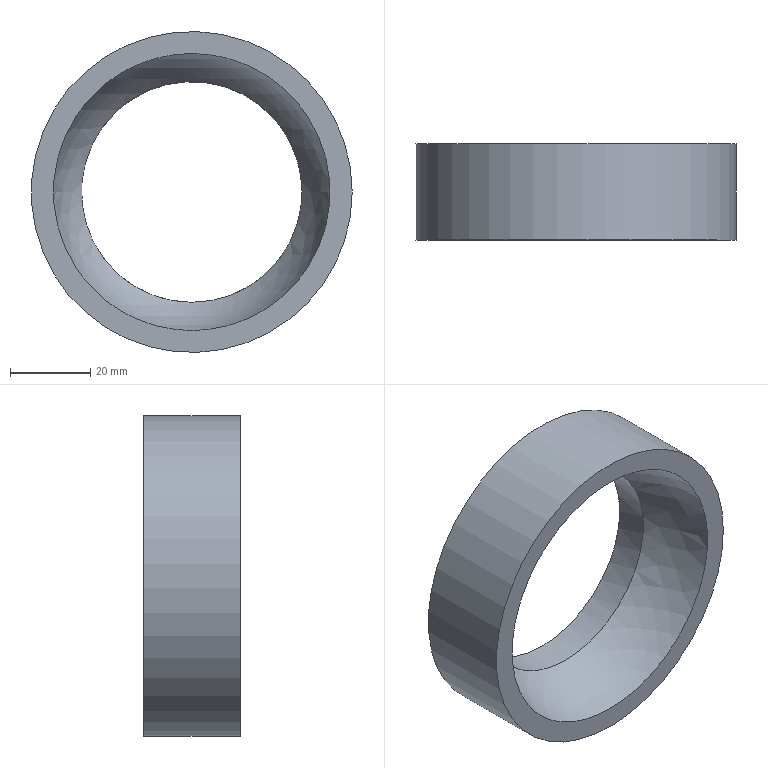Component | NX | MOVABLE_PAD | 1 solid | 5 faces | box 80 x 24 x 80 mm | volume 51017 mm3 | cylinder 2 | plane 2 | sphere 1 | commonest cylinder face diameters 80 x1 55 x1
STEP:
#1=CARTESIAN_POINT('',(0.,0.,0.));
#2=DIRECTION('',(0.,0.,1.));
#3=DIRECTION('',(1.,0.,0.));
#4=AXIS2_PLACEMENT_3D('',#1,#2,#3);
#5=CARTESIAN_POINT('',(223.939,30.,60.622));
#6=VERTEX_POINT('',#5);
#7=CARTESIAN_POINT('',(183.939,30.,60.622));
#8=DIRECTION('',(0.,-1.,0.));
#9=DIRECTION('',(1.,0.,0.));
#10=AXIS2_PLACEMENT_3D('',#7,#8,#9);
#11=CIRCLE('',#10,40.);
#12=CARTESIAN_POINT('',(183.939,30.,60.622));
#13=DIRECTION('',(0.,-1.,0.));
#14=DIRECTION('',(0.,0.,-1.));
#15=AXIS2_PLACEMENT_3D('',#12,#13,#14);
#16=CYLINDRICAL_SURFACE('',#15,40.);
#17=CARTESIAN_POINT('',(1.571,0.));
#18=DIRECTION('',(1.,0.));
#19=VECTOR('',#18,1.);
#20=LINE('',#17,#19);
#21=(GEOMETRIC_REPRESENTATION_CONTEXT(2)PARAMETRIC_REPRESENTATION_CONTEXT()REPRESENTATION_CONTEXT('',''));
#22=DEFINITIONAL_REPRESENTATION('',(#20),#21);
#23=PCURVE('',#16,#22);
#24=CARTESIAN_POINT('',(183.939,30.,60.622));
#25=DIRECTION('',(0.,-1.,0.));
#26=DIRECTION('',(0.,0.,-1.));
#27=AXIS2_PLACEMENT_3D('',#24,#25,#26);
#28=PLANE('',#27);
#29=CARTESIAN_POINT('',(0.,0.));
#30=DIRECTION('',(0.,1.));
#31=AXIS2_PLACEMENT_2D('',#29,#30);
#32=CIRCLE('',#31,40.);
#33=(GEOMETRIC_REPRESENTATION_CONTEXT(2)PARAMETRIC_REPRESENTATION_CONTEXT()REPRESENTATION_CONTEXT('',''));
#34=DEFINITIONAL_REPRESENTATION('',(#32),#33);
#35=PCURVE('',#28,#34);
#36=SURFACE_CURVE('',#11,(#23,#35),.PCURVE_S1.);
#37=EDGE_CURVE('',#6,#6,#36,.T.);
#38=ORIENTED_EDGE('',*,*,#37,.T.);
#39=CARTESIAN_POINT('',(223.939,6.,60.622));
#40=VERTEX_POINT('',#39);
#41=CARTESIAN_POINT('',(223.939,30.,60.622));
#42=CARTESIAN_POINT('',(223.939,6.,60.622));
#43=B_SPLINE_CURVE_WITH_KNOTS('',1,(#41,#42),.UNSPECIFIED.,.F.,.F.,(2,2),(0.,24.),.PIECEWISE_BEZIER_KNOTS.);
#44=CARTESIAN_POINT('',(7.854,0.));
#45=DIRECTION('',(0.,1.));
#46=VECTOR('',#45,1.);
#47=LINE('',#44,#46);
#48=(GEOMETRIC_REPRESENTATION_CONTEXT(2)PARAMETRIC_REPRESENTATION_CONTEXT()REPRESENTATION_CONTEXT('',''));
#49=DEFINITIONAL_REPRESENTATION('',(#47),#48);
#50=PCURVE('',#16,#49);
#51=CARTESIAN_POINT('',(1.571,0.));
#52=DIRECTION('',(0.,1.));
#53=VECTOR('',#52,1.);
#54=LINE('',#51,#53);
#55=(GEOMETRIC_REPRESENTATION_CONTEXT(2)PARAMETRIC_REPRESENTATION_CONTEXT()REPRESENTATION_CONTEXT('',''));
#56=DEFINITIONAL_REPRESENTATION('',(#54),#55);
#57=PCURVE('',#16,#56);
#58=SEAM_CURVE('',#43,(#50,#57),.PCURVE_S1.);
#59=EDGE_CURVE('',#6,#40,#58,.T.);
#60=ORIENTED_EDGE('',*,*,#59,.T.);
#61=CARTESIAN_POINT('',(183.939,6.,60.622));
#62=DIRECTION('',(0.,-1.,0.));
#63=DIRECTION('',(1.,0.,0.));
#64=AXIS2_PLACEMENT_3D('',#61,#62,#63);
#65=CIRCLE('',#64,40.);
#66=CARTESIAN_POINT('',(1.571,24.));
#67=DIRECTION('',(1.,0.));
#68=VECTOR('',#67,1.);
#69=LINE('',#66,#68);
#70=(GEOMETRIC_REPRESENTATION_CONTEXT(2)PARAMETRIC_REPRESENTATION_CONTEXT()REPRESENTATION_CONTEXT('',''));
#71=DEFINITIONAL_REPRESENTATION('',(#69),#70);
#72=PCURVE('',#16,#71);
#73=CARTESIAN_POINT('',(183.939,6.,60.622));
#74=DIRECTION('',(0.,-1.,0.));
#75=DIRECTION('',(0.,0.,-1.));
#76=AXIS2_PLACEMENT_3D('',#73,#74,#75);
#77=PLANE('',#76);
#78=CARTESIAN_POINT('',(0.,0.));
#79=DIRECTION('',(0.,1.));
#80=AXIS2_PLACEMENT_2D('',#78,#79);
#81=CIRCLE('',#80,40.);
#82=(GEOMETRIC_REPRESENTATION_CONTEXT(2)PARAMETRIC_REPRESENTATION_CONTEXT()REPRESENTATION_CONTEXT('',''));
#83=DEFINITIONAL_REPRESENTATION('',(#81),#82);
#84=PCURVE('',#77,#83);
#85=SURFACE_CURVE('',#65,(#72,#84),.PCURVE_S1.);
#86=EDGE_CURVE('',#40,#40,#85,.T.);
#87=ORIENTED_EDGE('',*,*,#86,.F.);
#88=ORIENTED_EDGE('',*,*,#59,.F.);
#89=EDGE_LOOP('',(#38,#60,#87,#88));
#90=FACE_BOUND('',#89,.T.);
#91=ADVANCED_FACE('',(#90),#16,.T.);
#92=CARTESIAN_POINT('',(183.939,21.651,33.122));
#93=VERTEX_POINT('',#92);
#94=CARTESIAN_POINT('',(183.939,21.651,60.622));
#95=DIRECTION('',(0.,-1.,0.));
#96=DIRECTION('',(0.,0.,-1.));
#97=AXIS2_PLACEMENT_3D('',#94,#95,#96);
#98=CIRCLE('',#97,27.5);
#99=CARTESIAN_POINT('',(183.939,30.,60.622));
#100=DIRECTION('',(0.,-1.,0.));
#101=DIRECTION('',(0.,0.,-1.));
#102=AXIS2_PLACEMENT_3D('',#99,#100,#101);
#103=CYLINDRICAL_SURFACE('',#102,27.5);
#104=CARTESIAN_POINT('',(0.,8.349));
#105=DIRECTION('',(1.,0.));
#106=VECTOR('',#105,1.);
#107=LINE('',#104,#106);
#108=(GEOMETRIC_REPRESENTATION_CONTEXT(2)PARAMETRIC_REPRESENTATION_CONTEXT()REPRESENTATION_CONTEXT('',''));
#109=DEFINITIONAL_REPRESENTATION('',(#107),#108);
#110=PCURVE('',#103,#109);
#111=CARTESIAN_POINT('',(183.939,-0.,60.622));
#112=DIRECTION('',(0.,0.,1.));
#113=DIRECTION('',(1.,0.,0.));
#114=AXIS2_PLACEMENT_3D('',#111,#112,#113);
#115=SPHERICAL_SURFACE('',#114,35.);
#116=CARTESIAN_POINT('',(1.571,-0.9038));
#117=CARTESIAN_POINT('',(1.443,-0.9044));
#118=CARTESIAN_POINT('',(1.213,-0.8677));
#119=CARTESIAN_POINT('',(0.9516,-0.7301));
#120=CARTESIAN_POINT('',(0.7946,-0.5446));
#121=CARTESIAN_POINT('',(0.7052,-0.3344));
#122=CARTESIAN_POINT('',(0.6653,-0.1126));
#123=CARTESIAN_POINT('',(0.6653,0.1126));
#124=CARTESIAN_POINT('',(0.7053,0.3344));
#125=CARTESIAN_POINT('',(0.7943,0.5446));
#126=CARTESIAN_POINT('',(0.9525,0.7301));
#127=CARTESIAN_POINT('',(1.21,0.868));
#128=CARTESIAN_POINT('',(1.571,0.9218));
#129=CARTESIAN_POINT('',(1.932,0.868));
#130=CARTESIAN_POINT('',(2.189,0.7301));
#131=CARTESIAN_POINT('',(2.347,0.5446));
#132=CARTESIAN_POINT('',(2.436,0.3344));
#133=CARTESIAN_POINT('',(2.476,0.1126));
#134=CARTESIAN_POINT('',(2.476,-0.1126));
#135=CARTESIAN_POINT('',(2.436,-0.3344));
#136=CARTESIAN_POINT('',(2.347,-0.5446));
#137=CARTESIAN_POINT('',(2.19,-0.7301));
#138=CARTESIAN_POINT('',(1.928,-0.8677));
#139=CARTESIAN_POINT('',(1.699,-0.9044));
#140=CARTESIAN_POINT('',(1.571,-0.9038));
#141=B_SPLINE_CURVE_WITH_KNOTS('',3,(#116,#117,#118,#119,#120,#121,#122,#123,#124,#125,#126,#127,#128,#129,#130,#131,#132,#133,#134,#135,#136,#137,#138,#139,#140),.UNSPECIFIED.,.T.,.F.,(4,1,1,1,1,1,1,1,1,1,1,1,1,1,1,1,1,1,1,1,1,1,4),(0.,0.2856,0.5712,0.8568,1.142,1.428,1.714,1.999,2.285,2.57,2.856,3.142,3.427,3.713,3.998,4.284,4.57,4.855,5.141,5.426,5.712,5.998,6.283),.QUASI_UNIFORM_KNOTS.);
#142=(GEOMETRIC_REPRESENTATION_CONTEXT(2)PARAMETRIC_REPRESENTATION_CONTEXT()REPRESENTATION_CONTEXT('',''));
#143=DEFINITIONAL_REPRESENTATION('',(#141),#142);
#144=PCURVE('',#115,#143);
#145=SURFACE_CURVE('',#98,(#110,#144),.PCURVE_S1.);
#146=EDGE_CURVE('',#93,#93,#145,.T.);
#147=ORIENTED_EDGE('',*,*,#146,.F.);
#148=CARTESIAN_POINT('',(183.939,30.,33.122));
#149=VERTEX_POINT('',#148);
#150=CARTESIAN_POINT('',(183.939,30.,33.122));
#151=CARTESIAN_POINT('',(183.939,21.651,33.122));
#152=B_SPLINE_CURVE_WITH_KNOTS('',1,(#150,#151),.UNSPECIFIED.,.F.,.F.,(2,2),(0.,8.349),.PIECEWISE_BEZIER_KNOTS.);
#153=CARTESIAN_POINT('',(0.,0.));
#154=DIRECTION('',(0.,1.));
#155=VECTOR('',#154,1.);
#156=LINE('',#153,#155);
#157=(GEOMETRIC_REPRESENTATION_CONTEXT(2)PARAMETRIC_REPRESENTATION_CONTEXT()REPRESENTATION_CONTEXT('',''));
#158=DEFINITIONAL_REPRESENTATION('',(#156),#157);
#159=PCURVE('',#103,#158);
#160=CARTESIAN_POINT('',(6.283,0.));
#161=DIRECTION('',(0.,1.));
#162=VECTOR('',#161,1.);
#163=LINE('',#160,#162);
#164=(GEOMETRIC_REPRESENTATION_CONTEXT(2)PARAMETRIC_REPRESENTATION_CONTEXT()REPRESENTATION_CONTEXT('',''));
#165=DEFINITIONAL_REPRESENTATION('',(#163),#164);
#166=PCURVE('',#103,#165);
#167=SEAM_CURVE('',#152,(#159,#166),.PCURVE_S1.);
#168=EDGE_CURVE('',#149,#93,#167,.T.);
#169=ORIENTED_EDGE('',*,*,#168,.F.);
#170=CARTESIAN_POINT('',(211.439,30.,60.622));
#171=VERTEX_POINT('',#170);
#172=CARTESIAN_POINT('',(183.939,30.,60.622));
#173=DIRECTION('',(0.,-1.,0.));
#174=DIRECTION('',(1.,0.,0.));
#175=AXIS2_PLACEMENT_3D('',#172,#173,#174);
#176=CIRCLE('',#175,27.5);
#177=CARTESIAN_POINT('',(-4.712,0.));
#178=DIRECTION('',(1.,0.));
#179=VECTOR('',#178,1.);
#180=LINE('',#177,#179);
#181=(GEOMETRIC_REPRESENTATION_CONTEXT(2)PARAMETRIC_REPRESENTATION_CONTEXT()REPRESENTATION_CONTEXT('',''));
#182=DEFINITIONAL_REPRESENTATION('',(#180),#181);
#183=PCURVE('',#103,#182);
#184=CARTESIAN_POINT('',(0.,0.));
#185=DIRECTION('',(0.,1.));
#186=AXIS2_PLACEMENT_2D('',#184,#185);
#187=CIRCLE('',#186,27.5);
#188=(GEOMETRIC_REPRESENTATION_CONTEXT(2)PARAMETRIC_REPRESENTATION_CONTEXT()REPRESENTATION_CONTEXT('',''));
#189=DEFINITIONAL_REPRESENTATION('',(#187),#188);
#190=PCURVE('',#28,#189);
#191=SURFACE_CURVE('',#176,(#183,#190),.PCURVE_S1.);
#192=EDGE_CURVE('',#149,#171,#191,.T.);
#193=ORIENTED_EDGE('',*,*,#192,.T.);
#194=CARTESIAN_POINT('',(183.939,30.,60.622));
#195=DIRECTION('',(0.,-1.,0.));
#196=DIRECTION('',(1.,0.,0.));
#197=AXIS2_PLACEMENT_3D('',#194,#195,#196);
#198=CIRCLE('',#197,27.5);
#199=CARTESIAN_POINT('',(1.571,0.));
#200=DIRECTION('',(1.,0.));
#201=VECTOR('',#200,1.);
#202=LINE('',#199,#201);
#203=(GEOMETRIC_REPRESENTATION_CONTEXT(2)PARAMETRIC_REPRESENTATION_CONTEXT()REPRESENTATION_CONTEXT('',''));
#204=DEFINITIONAL_REPRESENTATION('',(#202),#203);
#205=PCURVE('',#103,#204);
#206=CARTESIAN_POINT('',(0.,0.));
#207=DIRECTION('',(0.,1.));
#208=AXIS2_PLACEMENT_2D('',#206,#207);
#209=CIRCLE('',#208,27.5);
#210=(GEOMETRIC_REPRESENTATION_CONTEXT(2)PARAMETRIC_REPRESENTATION_CONTEXT()REPRESENTATION_CONTEXT('',''));
#211=DEFINITIONAL_REPRESENTATION('',(#209),#210);
#212=PCURVE('',#28,#211);
#213=SURFACE_CURVE('',#198,(#205,#212),.PCURVE_S1.);
#214=EDGE_CURVE('',#171,#149,#213,.T.);
#215=ORIENTED_EDGE('',*,*,#214,.T.);
#216=ORIENTED_EDGE('',*,*,#168,.T.);
#217=EDGE_LOOP('',(#147,#169,#193,#215,#216));
#218=FACE_BOUND('',#217,.F.);
#219=ADVANCED_FACE('',(#218),#103,.F.);
#220=ORIENTED_EDGE('',*,*,#37,.F.);
#221=EDGE_LOOP('',(#220));
#222=FACE_BOUND('',#221,.T.);
#223=ORIENTED_EDGE('',*,*,#214,.T.);
#224=ORIENTED_EDGE('',*,*,#192,.T.);
#225=EDGE_LOOP('',(#223,#224));
#226=FACE_BOUND('',#225,.T.);
#227=ADVANCED_FACE('',(#222,#226),#28,.F.);
#228=CARTESIAN_POINT('',(183.939,6.,26.14));
#229=VERTEX_POINT('',#228);
#230=CARTESIAN_POINT('',(183.939,6.,60.622));
#231=DIRECTION('',(0.,-1.,0.));
#232=DIRECTION('',(0.,0.,-1.));
#233=AXIS2_PLACEMENT_3D('',#230,#231,#232);
#234=CIRCLE('',#233,34.482);
#235=CARTESIAN_POINT('',(0.,0.));
#236=DIRECTION('',(1.,0.));
#237=AXIS2_PLACEMENT_2D('',#235,#236);
#238=CIRCLE('',#237,34.482);
#239=(GEOMETRIC_REPRESENTATION_CONTEXT(2)PARAMETRIC_REPRESENTATION_CONTEXT()REPRESENTATION_CONTEXT('',''));
#240=DEFINITIONAL_REPRESENTATION('',(#238),#239);
#241=PCURVE('',#77,#240);
#242=CARTESIAN_POINT('',(1.571,-1.399));
#243=CARTESIAN_POINT('',(1.034,-1.372));
#244=CARTESIAN_POINT('',(0.4173,-1.256));
#245=CARTESIAN_POINT('',(0.3089,-0.9757));
#246=CARTESIAN_POINT('',(0.2155,-0.7025));
#247=CARTESIAN_POINT('',(0.1867,-0.4216));
#248=CARTESIAN_POINT('',(0.1716,-0.1408));
#249=CARTESIAN_POINT('',(0.1712,0.1407));
#250=CARTESIAN_POINT('',(0.1879,0.4219));
#251=CARTESIAN_POINT('',(0.2111,0.7016));
#252=CARTESIAN_POINT('',(0.3253,0.979));
#253=CARTESIAN_POINT('',(0.3559,1.244));
#254=CARTESIAN_POINT('',(1.571,1.476));
#255=CARTESIAN_POINT('',(2.786,1.244));
#256=CARTESIAN_POINT('',(2.816,0.979));
#257=CARTESIAN_POINT('',(2.93,0.7016));
#258=CARTESIAN_POINT('',(2.954,0.4219));
#259=CARTESIAN_POINT('',(2.97,0.1407));
#260=CARTESIAN_POINT('',(2.97,-0.1408));
#261=CARTESIAN_POINT('',(2.955,-0.4216));
#262=CARTESIAN_POINT('',(2.926,-0.7025));
#263=CARTESIAN_POINT('',(2.833,-0.9757));
#264=CARTESIAN_POINT('',(2.724,-1.256));
#265=CARTESIAN_POINT('',(2.108,-1.372));
#266=CARTESIAN_POINT('',(1.571,-1.399));
#267=B_SPLINE_CURVE_WITH_KNOTS('',3,(#242,#243,#244,#245,#246,#247,#248,#249,#250,#251,#252,#253,#254,#255,#256,#257,#258,#259,#260,#261,#262,#263,#264,#265,#266),.UNSPECIFIED.,.T.,.F.,(4,1,1,1,1,1,1,1,1,1,1,1,1,1,1,1,1,1,1,1,1,1,4),(0.,0.2856,0.5712,0.8568,1.142,1.428,1.714,1.999,2.285,2.57,2.856,3.142,3.427,3.713,3.998,4.284,4.57,4.855,5.141,5.426,5.712,5.998,6.283),.QUASI_UNIFORM_KNOTS.);
#268=(GEOMETRIC_REPRESENTATION_CONTEXT(2)PARAMETRIC_REPRESENTATION_CONTEXT()REPRESENTATION_CONTEXT('',''));
#269=DEFINITIONAL_REPRESENTATION('',(#267),#268);
#270=PCURVE('',#115,#269);
#271=SURFACE_CURVE('',#234,(#241,#270),.PCURVE_S1.);
#272=EDGE_CURVE('',#229,#229,#271,.T.);
#273=ORIENTED_EDGE('',*,*,#272,.F.);
#274=EDGE_LOOP('',(#273));
#275=FACE_BOUND('',#274,.T.);
#276=ORIENTED_EDGE('',*,*,#86,.T.);
#277=EDGE_LOOP('',(#276));
#278=FACE_BOUND('',#277,.T.);
#279=ADVANCED_FACE('',(#275,#278),#77,.T.);
#280=ORIENTED_EDGE('',*,*,#272,.F.);
#281=EDGE_LOOP('',(#280));
#282=FACE_BOUND('',#281,.F.);
#283=ORIENTED_EDGE('',*,*,#146,.T.);
#284=EDGE_LOOP('',(#283));
#285=FACE_BOUND('',#284,.F.);
#286=ADVANCED_FACE('',(#282,#285),#115,.F.);
#287=CLOSED_SHELL('',(#91,#219,#227,#279,#286));
#288=MANIFOLD_SOLID_BREP('',#287);
#289=(LENGTH_UNIT()NAMED_UNIT(*)SI_UNIT(.MILLI.,.METRE.));
#290=UNCERTAINTY_MEASURE_WITH_UNIT(LENGTH_MEASURE(0.000005),#289,'','');
#291=(NAMED_UNIT(*)PLANE_ANGLE_UNIT()SI_UNIT($,.RADIAN.));
#292=(NAMED_UNIT(*)SI_UNIT($,.STERADIAN.)SOLID_ANGLE_UNIT());
#293=(GEOMETRIC_REPRESENTATION_CONTEXT(3)GLOBAL_UNCERTAINTY_ASSIGNED_CONTEXT((#290))GLOBAL_UNIT_ASSIGNED_CONTEXT((#289,#291,#292))REPRESENTATION_CONTEXT('',''));
#294=ADVANCED_BREP_SHAPE_REPRESENTATION('',(#4,#288),#293);